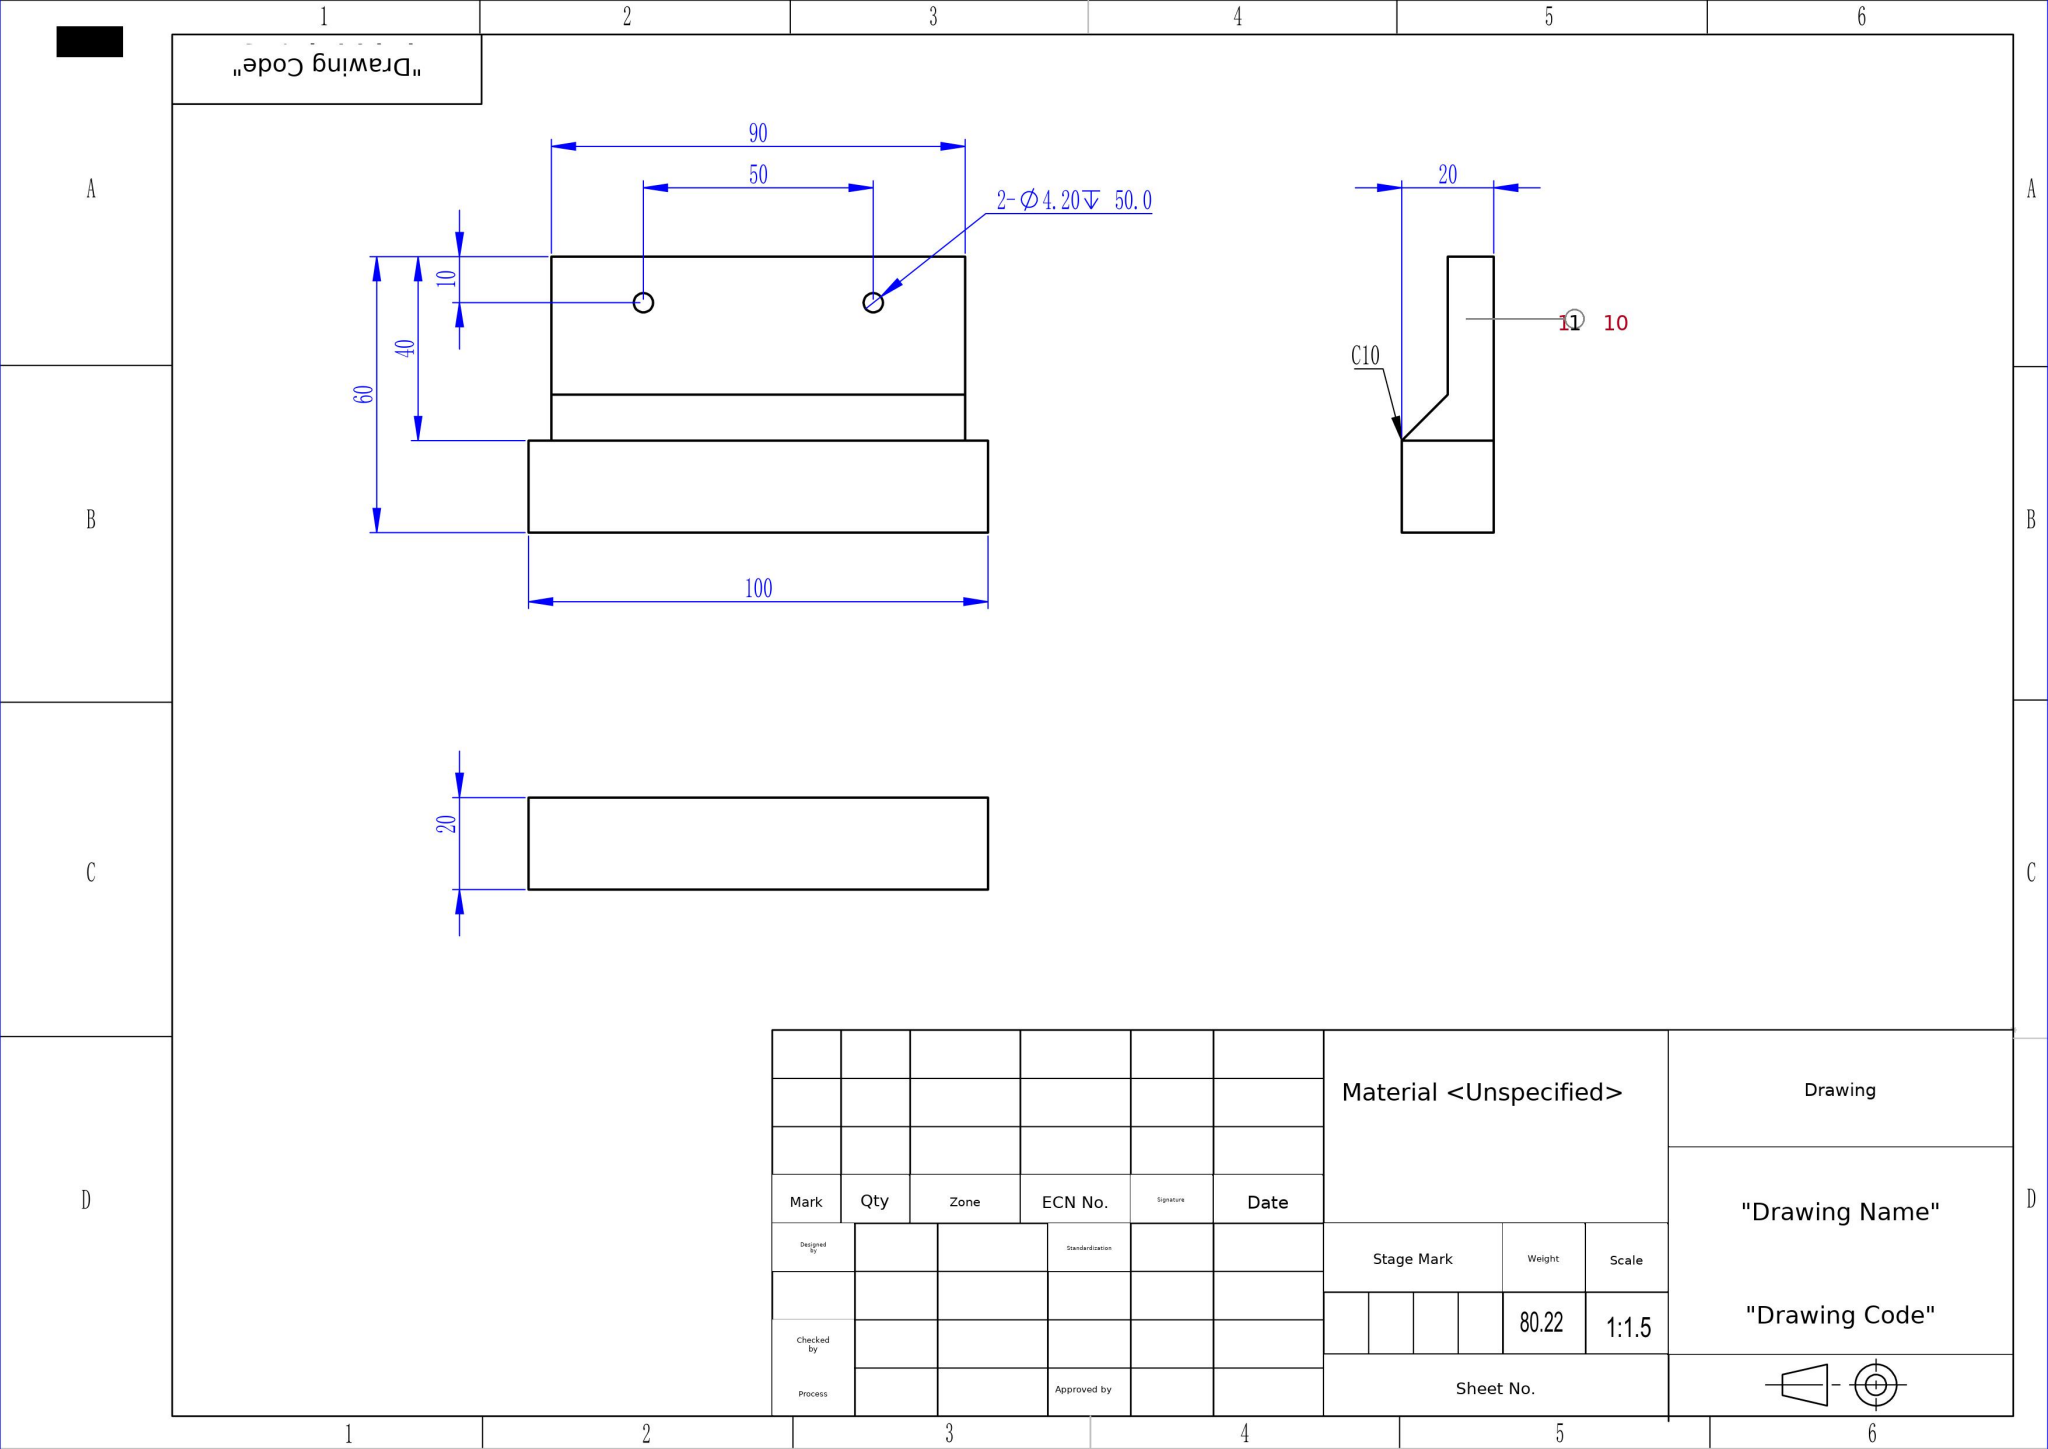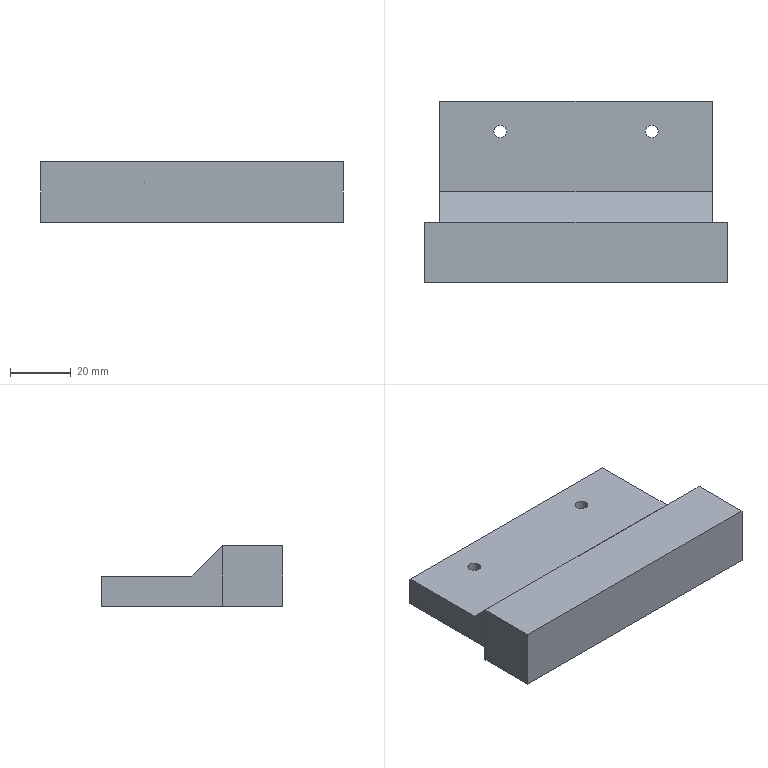Part | SolidWorks | mm | material Unspecified | 1 solid | 16 faces | box 100 x 60 x 20 mm | volume 80223 mm3 | plane 12 | cylinder 4 | commonest cylinder face diameters 4.2 x4
STEP:
#1=CARTESIAN_POINT('',(-27.1,40.,-10.));
#2=VERTEX_POINT('',#1);
#3=CARTESIAN_POINT('',(-22.9,40.,-10.));
#4=VERTEX_POINT('',#3);
#5=CARTESIAN_POINT('',(-25.,40.,-10.));
#6=DIRECTION('',(0.,0.,1.));
#7=DIRECTION('',(1.,0.,0.));
#8=AXIS2_PLACEMENT_3D('',#5,#6,#7);
#9=CIRCLE('',#8,2.1);
#10=EDGE_CURVE('',#2,#4,#9,.T.);
#11=ORIENTED_EDGE('',*,*,#10,.F.);
#12=CARTESIAN_POINT('',(-27.1,40.,0.));
#13=VERTEX_POINT('',#12);
#14=CARTESIAN_POINT('',(-27.1,40.,-50.));
#15=DIRECTION('',(0.,0.,1.));
#16=VECTOR('',#15,1000.);
#17=LINE('',#14,#16);
#18=EDGE_CURVE('',#2,#13,#17,.T.);
#19=ORIENTED_EDGE('',*,*,#18,.T.);
#20=CARTESIAN_POINT('',(-22.9,40.,0.));
#21=VERTEX_POINT('',#20);
#22=CARTESIAN_POINT('',(-25.,40.,0.));
#23=DIRECTION('',(0.,0.,1.));
#24=DIRECTION('',(1.,0.,0.));
#25=AXIS2_PLACEMENT_3D('',#22,#23,#24);
#26=CIRCLE('',#25,2.1);
#27=EDGE_CURVE('',#13,#21,#26,.T.);
#28=ORIENTED_EDGE('',*,*,#27,.T.);
#29=CARTESIAN_POINT('',(-22.9,40.,-50.));
#30=DIRECTION('',(0.,0.,1.));
#31=VECTOR('',#30,1000.);
#32=LINE('',#29,#31);
#33=EDGE_CURVE('',#4,#21,#32,.T.);
#34=ORIENTED_EDGE('',*,*,#33,.F.);
#35=EDGE_LOOP('',(#11,#19,#28,#34));
#36=FACE_OUTER_BOUND('',#35,.T.);
#37=CARTESIAN_POINT('',(-25.,40.,-50.));
#38=DIRECTION('',(0.,0.,1.));
#39=DIRECTION('',(1.,0.,0.));
#40=AXIS2_PLACEMENT_3D('',#37,#38,#39);
#41=CYLINDRICAL_SURFACE('',#40,2.1);
#42=ADVANCED_FACE('',(#36),#41,.F.);
#43=CARTESIAN_POINT('',(22.9,40.,-10.));
#44=VERTEX_POINT('',#43);
#45=CARTESIAN_POINT('',(27.1,40.,-10.));
#46=VERTEX_POINT('',#45);
#47=CARTESIAN_POINT('',(25.,40.,-10.));
#48=DIRECTION('',(0.,0.,1.));
#49=DIRECTION('',(1.,0.,0.));
#50=AXIS2_PLACEMENT_3D('',#47,#48,#49);
#51=CIRCLE('',#50,2.1);
#52=EDGE_CURVE('',#44,#46,#51,.T.);
#53=ORIENTED_EDGE('',*,*,#52,.F.);
#54=CARTESIAN_POINT('',(22.9,40.,0.));
#55=VERTEX_POINT('',#54);
#56=CARTESIAN_POINT('',(22.9,40.,-50.));
#57=DIRECTION('',(0.,0.,1.));
#58=VECTOR('',#57,1000.);
#59=LINE('',#56,#58);
#60=EDGE_CURVE('',#44,#55,#59,.T.);
#61=ORIENTED_EDGE('',*,*,#60,.T.);
#62=CARTESIAN_POINT('',(27.1,40.,0.));
#63=VERTEX_POINT('',#62);
#64=CARTESIAN_POINT('',(25.,40.,0.));
#65=DIRECTION('',(0.,0.,1.));
#66=DIRECTION('',(1.,0.,0.));
#67=AXIS2_PLACEMENT_3D('',#64,#65,#66);
#68=CIRCLE('',#67,2.1);
#69=EDGE_CURVE('',#55,#63,#68,.T.);
#70=ORIENTED_EDGE('',*,*,#69,.T.);
#71=CARTESIAN_POINT('',(27.1,40.,-50.));
#72=DIRECTION('',(0.,0.,1.));
#73=VECTOR('',#72,1000.);
#74=LINE('',#71,#73);
#75=EDGE_CURVE('',#46,#63,#74,.T.);
#76=ORIENTED_EDGE('',*,*,#75,.F.);
#77=EDGE_LOOP('',(#53,#61,#70,#76));
#78=FACE_OUTER_BOUND('',#77,.T.);
#79=CARTESIAN_POINT('',(25.,40.,-50.));
#80=DIRECTION('',(0.,0.,1.));
#81=DIRECTION('',(1.,0.,0.));
#82=AXIS2_PLACEMENT_3D('',#79,#80,#81);
#83=CYLINDRICAL_SURFACE('',#82,2.1);
#84=ADVANCED_FACE('',(#78),#83,.F.);
#85=CARTESIAN_POINT('',(45.,10.,10.));
#86=VERTEX_POINT('',#85);
#87=CARTESIAN_POINT('',(45.,10.,-10.));
#88=VERTEX_POINT('',#87);
#89=CARTESIAN_POINT('',(45.,10.,-10.));
#90=DIRECTION('',(0.,0.,-1.));
#91=VECTOR('',#90,1000.);
#92=LINE('',#89,#91);
#93=EDGE_CURVE('',#86,#88,#92,.T.);
#94=ORIENTED_EDGE('',*,*,#93,.F.);
#95=CARTESIAN_POINT('',(50.,10.,10.));
#96=VERTEX_POINT('',#95);
#97=CARTESIAN_POINT('',(-50.,10.,10.));
#98=DIRECTION('',(-1.,0.,0.));
#99=VECTOR('',#98,1000.);
#100=LINE('',#97,#99);
#101=EDGE_CURVE('',#96,#86,#100,.T.);
#102=ORIENTED_EDGE('',*,*,#101,.F.);
#103=CARTESIAN_POINT('',(50.,10.,-10.));
#104=VERTEX_POINT('',#103);
#105=CARTESIAN_POINT('',(50.,10.,-10.));
#106=DIRECTION('',(0.,0.,1.));
#107=VECTOR('',#106,1000.);
#108=LINE('',#105,#107);
#109=EDGE_CURVE('',#104,#96,#108,.T.);
#110=ORIENTED_EDGE('',*,*,#109,.F.);
#111=CARTESIAN_POINT('',(-50.,10.,-10.));
#112=DIRECTION('',(-1.,0.,0.));
#113=VECTOR('',#112,1000.);
#114=LINE('',#111,#113);
#115=EDGE_CURVE('',#104,#88,#114,.T.);
#116=ORIENTED_EDGE('',*,*,#115,.T.);
#117=EDGE_LOOP('',(#94,#102,#110,#116));
#118=FACE_OUTER_BOUND('',#117,.T.);
#119=CARTESIAN_POINT('',(-50.,10.,-10.));
#120=DIRECTION('',(0.,1.,0.));
#121=DIRECTION('',(0.,0.,1.));
#122=AXIS2_PLACEMENT_3D('',#119,#120,#121);
#123=PLANE('',#122);
#124=ADVANCED_FACE('',(#118),#123,.T.);
#125=ORIENTED_EDGE('',*,*,#109,.T.);
#126=CARTESIAN_POINT('',(50.,-10.,10.));
#127=VERTEX_POINT('',#126);
#128=CARTESIAN_POINT('',(50.,10.,10.));
#129=DIRECTION('',(0.,1.,0.));
#130=VECTOR('',#129,1000.);
#131=LINE('',#128,#130);
#132=EDGE_CURVE('',#127,#96,#131,.T.);
#133=ORIENTED_EDGE('',*,*,#132,.F.);
#134=CARTESIAN_POINT('',(50.,-10.,-10.));
#135=VERTEX_POINT('',#134);
#136=CARTESIAN_POINT('',(50.,-10.,-10.));
#137=DIRECTION('',(0.,0.,1.));
#138=VECTOR('',#137,1000.);
#139=LINE('',#136,#138);
#140=EDGE_CURVE('',#135,#127,#139,.T.);
#141=ORIENTED_EDGE('',*,*,#140,.F.);
#142=CARTESIAN_POINT('',(50.,10.,-10.));
#143=DIRECTION('',(0.,1.,0.));
#144=VECTOR('',#143,1000.);
#145=LINE('',#142,#144);
#146=EDGE_CURVE('',#135,#104,#145,.T.);
#147=ORIENTED_EDGE('',*,*,#146,.T.);
#148=EDGE_LOOP('',(#125,#133,#141,#147));
#149=FACE_OUTER_BOUND('',#148,.T.);
#150=CARTESIAN_POINT('',(50.,10.,-10.));
#151=DIRECTION('',(1.,0.,0.));
#152=DIRECTION('',(0.,0.,-1.));
#153=AXIS2_PLACEMENT_3D('',#150,#151,#152);
#154=PLANE('',#153);
#155=ADVANCED_FACE('',(#149),#154,.T.);
#156=ORIENTED_EDGE('',*,*,#140,.T.);
#157=CARTESIAN_POINT('',(-50.,-10.,10.));
#158=VERTEX_POINT('',#157);
#159=CARTESIAN_POINT('',(-50.,-10.,10.));
#160=DIRECTION('',(1.,0.,0.));
#161=VECTOR('',#160,1000.);
#162=LINE('',#159,#161);
#163=EDGE_CURVE('',#158,#127,#162,.T.);
#164=ORIENTED_EDGE('',*,*,#163,.F.);
#165=CARTESIAN_POINT('',(-50.,-10.,-10.));
#166=VERTEX_POINT('',#165);
#167=CARTESIAN_POINT('',(-50.,-10.,-10.));
#168=DIRECTION('',(0.,0.,1.));
#169=VECTOR('',#168,1000.);
#170=LINE('',#167,#169);
#171=EDGE_CURVE('',#166,#158,#170,.T.);
#172=ORIENTED_EDGE('',*,*,#171,.F.);
#173=CARTESIAN_POINT('',(-50.,-10.,-10.));
#174=DIRECTION('',(1.,0.,0.));
#175=VECTOR('',#174,1000.);
#176=LINE('',#173,#175);
#177=EDGE_CURVE('',#166,#135,#176,.T.);
#178=ORIENTED_EDGE('',*,*,#177,.T.);
#179=EDGE_LOOP('',(#156,#164,#172,#178));
#180=FACE_OUTER_BOUND('',#179,.T.);
#181=CARTESIAN_POINT('',(-50.,-10.,-10.));
#182=DIRECTION('',(0.,-1.,0.));
#183=DIRECTION('',(0.,0.,-1.));
#184=AXIS2_PLACEMENT_3D('',#181,#182,#183);
#185=PLANE('',#184);
#186=ADVANCED_FACE('',(#180),#185,.T.);
#187=ORIENTED_EDGE('',*,*,#171,.T.);
#188=CARTESIAN_POINT('',(-50.,10.,10.));
#189=VERTEX_POINT('',#188);
#190=CARTESIAN_POINT('',(-50.,10.,10.));
#191=DIRECTION('',(0.,-1.,0.));
#192=VECTOR('',#191,1000.);
#193=LINE('',#190,#192);
#194=EDGE_CURVE('',#189,#158,#193,.T.);
#195=ORIENTED_EDGE('',*,*,#194,.F.);
#196=CARTESIAN_POINT('',(-50.,10.,-10.));
#197=VERTEX_POINT('',#196);
#198=CARTESIAN_POINT('',(-50.,10.,-10.));
#199=DIRECTION('',(0.,0.,1.));
#200=VECTOR('',#199,1000.);
#201=LINE('',#198,#200);
#202=EDGE_CURVE('',#197,#189,#201,.T.);
#203=ORIENTED_EDGE('',*,*,#202,.F.);
#204=CARTESIAN_POINT('',(-50.,10.,-10.));
#205=DIRECTION('',(0.,-1.,0.));
#206=VECTOR('',#205,1000.);
#207=LINE('',#204,#206);
#208=EDGE_CURVE('',#197,#166,#207,.T.);
#209=ORIENTED_EDGE('',*,*,#208,.T.);
#210=EDGE_LOOP('',(#187,#195,#203,#209));
#211=FACE_OUTER_BOUND('',#210,.T.);
#212=CARTESIAN_POINT('',(-50.,10.,-10.));
#213=DIRECTION('',(-1.,0.,0.));
#214=DIRECTION('',(0.,0.,1.));
#215=AXIS2_PLACEMENT_3D('',#212,#213,#214);
#216=PLANE('',#215);
#217=ADVANCED_FACE('',(#211),#216,.T.);
#218=CARTESIAN_POINT('',(-45.,10.,10.));
#219=VERTEX_POINT('',#218);
#220=CARTESIAN_POINT('',(-50.,10.,10.));
#221=DIRECTION('',(-1.,0.,0.));
#222=VECTOR('',#221,1000.);
#223=LINE('',#220,#222);
#224=EDGE_CURVE('',#219,#189,#223,.T.);
#225=ORIENTED_EDGE('',*,*,#224,.F.);
#226=CARTESIAN_POINT('',(-45.,10.,-10.));
#227=VERTEX_POINT('',#226);
#228=CARTESIAN_POINT('',(-45.,10.,-10.));
#229=DIRECTION('',(0.,0.,1.));
#230=VECTOR('',#229,1000.);
#231=LINE('',#228,#230);
#232=EDGE_CURVE('',#227,#219,#231,.T.);
#233=ORIENTED_EDGE('',*,*,#232,.F.);
#234=CARTESIAN_POINT('',(-50.,10.,-10.));
#235=DIRECTION('',(-1.,0.,0.));
#236=VECTOR('',#235,1000.);
#237=LINE('',#234,#236);
#238=EDGE_CURVE('',#227,#197,#237,.T.);
#239=ORIENTED_EDGE('',*,*,#238,.T.);
#240=ORIENTED_EDGE('',*,*,#202,.T.);
#241=EDGE_LOOP('',(#225,#233,#239,#240));
#242=FACE_OUTER_BOUND('',#241,.T.);
#243=CARTESIAN_POINT('',(-50.,10.,-10.));
#244=DIRECTION('',(0.,1.,0.));
#245=DIRECTION('',(0.,0.,1.));
#246=AXIS2_PLACEMENT_3D('',#243,#244,#245);
#247=PLANE('',#246);
#248=ADVANCED_FACE('',(#242),#247,.T.);
#249=CARTESIAN_POINT('',(-25.,40.,-10.));
#250=DIRECTION('',(0.,0.,1.));
#251=DIRECTION('',(1.,0.,0.));
#252=AXIS2_PLACEMENT_3D('',#249,#250,#251);
#253=CIRCLE('',#252,2.1);
#254=EDGE_CURVE('',#4,#2,#253,.T.);
#255=ORIENTED_EDGE('',*,*,#254,.T.);
#256=ORIENTED_EDGE('',*,*,#10,.T.);
#257=EDGE_LOOP('',(#255,#256));
#258=FACE_BOUND('',#257,.T.);
#259=CARTESIAN_POINT('',(25.,40.,-10.));
#260=DIRECTION('',(0.,0.,1.));
#261=DIRECTION('',(1.,0.,0.));
#262=AXIS2_PLACEMENT_3D('',#259,#260,#261);
#263=CIRCLE('',#262,2.1);
#264=EDGE_CURVE('',#46,#44,#263,.T.);
#265=ORIENTED_EDGE('',*,*,#264,.T.);
#266=ORIENTED_EDGE('',*,*,#52,.T.);
#267=EDGE_LOOP('',(#265,#266));
#268=FACE_BOUND('',#267,.T.);
#269=CARTESIAN_POINT('',(-45.,50.,-10.));
#270=VERTEX_POINT('',#269);
#271=CARTESIAN_POINT('',(-45.,60.,-10.));
#272=DIRECTION('',(0.,-1.,0.));
#273=VECTOR('',#272,1000.);
#274=LINE('',#271,#273);
#275=EDGE_CURVE('',#270,#227,#274,.T.);
#276=ORIENTED_EDGE('',*,*,#275,.F.);
#277=CARTESIAN_POINT('',(45.,50.,-10.));
#278=VERTEX_POINT('',#277);
#279=CARTESIAN_POINT('',(0.,50.,-10.));
#280=DIRECTION('',(1.,0.,0.));
#281=VECTOR('',#280,1000.);
#282=LINE('',#279,#281);
#283=EDGE_CURVE('',#270,#278,#282,.T.);
#284=ORIENTED_EDGE('',*,*,#283,.T.);
#285=CARTESIAN_POINT('',(45.,60.,-10.));
#286=DIRECTION('',(0.,-1.,0.));
#287=VECTOR('',#286,1000.);
#288=LINE('',#285,#287);
#289=EDGE_CURVE('',#278,#88,#288,.T.);
#290=ORIENTED_EDGE('',*,*,#289,.T.);
#291=ORIENTED_EDGE('',*,*,#115,.F.);
#292=ORIENTED_EDGE('',*,*,#146,.F.);
#293=ORIENTED_EDGE('',*,*,#177,.F.);
#294=ORIENTED_EDGE('',*,*,#208,.F.);
#295=ORIENTED_EDGE('',*,*,#238,.F.);
#296=EDGE_LOOP('',(#276,#284,#290,#291,#292,#293,#294,#295));
#297=FACE_OUTER_BOUND('',#296,.T.);
#298=CARTESIAN_POINT('',(0.,0.,-10.));
#299=DIRECTION('',(0.,0.,1.));
#300=DIRECTION('',(1.,0.,0.));
#301=AXIS2_PLACEMENT_3D('',#298,#299,#300);
#302=PLANE('',#301);
#303=ADVANCED_FACE('',(#258,#268,#297),#302,.F.);
#304=ORIENTED_EDGE('',*,*,#132,.T.);
#305=ORIENTED_EDGE('',*,*,#101,.T.);
#306=CARTESIAN_POINT('',(-50.,10.,10.));
#307=DIRECTION('',(-1.,0.,0.));
#308=VECTOR('',#307,1000.);
#309=LINE('',#306,#308);
#310=EDGE_CURVE('',#86,#219,#309,.T.);
#311=ORIENTED_EDGE('',*,*,#310,.T.);
#312=ORIENTED_EDGE('',*,*,#224,.T.);
#313=ORIENTED_EDGE('',*,*,#194,.T.);
#314=ORIENTED_EDGE('',*,*,#163,.T.);
#315=EDGE_LOOP('',(#304,#305,#311,#312,#313,#314));
#316=FACE_OUTER_BOUND('',#315,.T.);
#317=CARTESIAN_POINT('',(0.,0.,10.));
#318=DIRECTION('',(0.,0.,1.));
#319=DIRECTION('',(1.,0.,0.));
#320=AXIS2_PLACEMENT_3D('',#317,#318,#319);
#321=PLANE('',#320);
#322=ADVANCED_FACE('',(#316),#321,.T.);
#323=CARTESIAN_POINT('',(-45.,50.,0.));
#324=VERTEX_POINT('',#323);
#325=CARTESIAN_POINT('',(-45.,20.,0.));
#326=VERTEX_POINT('',#325);
#327=CARTESIAN_POINT('',(-45.,60.,0.));
#328=DIRECTION('',(0.,-1.,0.));
#329=VECTOR('',#328,1000.);
#330=LINE('',#327,#329);
#331=EDGE_CURVE('',#324,#326,#330,.T.);
#332=ORIENTED_EDGE('',*,*,#331,.F.);
#333=CARTESIAN_POINT('',(-45.,50.,-50.));
#334=DIRECTION('',(0.,0.,1.));
#335=VECTOR('',#334,1000.);
#336=LINE('',#333,#335);
#337=EDGE_CURVE('',#270,#324,#336,.T.);
#338=ORIENTED_EDGE('',*,*,#337,.F.);
#339=ORIENTED_EDGE('',*,*,#275,.T.);
#340=ORIENTED_EDGE('',*,*,#232,.T.);
#341=CARTESIAN_POINT('',(-45.,45.,-25.));
#342=DIRECTION('',(0.,0.7071,-0.7071));
#343=VECTOR('',#342,1000.);
#344=LINE('',#341,#343);
#345=EDGE_CURVE('',#219,#326,#344,.T.);
#346=ORIENTED_EDGE('',*,*,#345,.T.);
#347=EDGE_LOOP('',(#332,#338,#339,#340,#346));
#348=FACE_OUTER_BOUND('',#347,.T.);
#349=CARTESIAN_POINT('',(-45.,60.,-10.));
#350=DIRECTION('',(1.,0.,0.));
#351=DIRECTION('',(0.,0.,-1.));
#352=AXIS2_PLACEMENT_3D('',#349,#350,#351);
#353=PLANE('',#352);
#354=ADVANCED_FACE('',(#348),#353,.F.);
#355=CARTESIAN_POINT('',(-25.,40.,0.));
#356=DIRECTION('',(0.,0.,1.));
#357=DIRECTION('',(1.,0.,0.));
#358=AXIS2_PLACEMENT_3D('',#355,#356,#357);
#359=CIRCLE('',#358,2.1);
#360=EDGE_CURVE('',#21,#13,#359,.T.);
#361=ORIENTED_EDGE('',*,*,#360,.F.);
#362=ORIENTED_EDGE('',*,*,#27,.F.);
#363=EDGE_LOOP('',(#361,#362));
#364=FACE_BOUND('',#363,.T.);
#365=CARTESIAN_POINT('',(25.,40.,0.));
#366=DIRECTION('',(0.,0.,1.));
#367=DIRECTION('',(1.,0.,0.));
#368=AXIS2_PLACEMENT_3D('',#365,#366,#367);
#369=CIRCLE('',#368,2.1);
#370=EDGE_CURVE('',#63,#55,#369,.T.);
#371=ORIENTED_EDGE('',*,*,#370,.F.);
#372=ORIENTED_EDGE('',*,*,#69,.F.);
#373=EDGE_LOOP('',(#371,#372));
#374=FACE_BOUND('',#373,.T.);
#375=CARTESIAN_POINT('',(45.,50.,0.));
#376=VERTEX_POINT('',#375);
#377=CARTESIAN_POINT('',(45.,20.,0.));
#378=VERTEX_POINT('',#377);
#379=CARTESIAN_POINT('',(45.,60.,0.));
#380=DIRECTION('',(0.,-1.,0.));
#381=VECTOR('',#380,1000.);
#382=LINE('',#379,#381);
#383=EDGE_CURVE('',#376,#378,#382,.T.);
#384=ORIENTED_EDGE('',*,*,#383,.F.);
#385=CARTESIAN_POINT('',(-45.,50.,0.));
#386=DIRECTION('',(1.,0.,0.));
#387=VECTOR('',#386,1000.);
#388=LINE('',#385,#387);
#389=EDGE_CURVE('',#324,#376,#388,.T.);
#390=ORIENTED_EDGE('',*,*,#389,.F.);
#391=ORIENTED_EDGE('',*,*,#331,.T.);
#392=CARTESIAN_POINT('',(-45.,20.,0.));
#393=DIRECTION('',(1.,0.,0.));
#394=VECTOR('',#393,1000.);
#395=LINE('',#392,#394);
#396=EDGE_CURVE('',#326,#378,#395,.T.);
#397=ORIENTED_EDGE('',*,*,#396,.T.);
#398=EDGE_LOOP('',(#384,#390,#391,#397));
#399=FACE_OUTER_BOUND('',#398,.T.);
#400=CARTESIAN_POINT('',(-45.,60.,0.));
#401=DIRECTION('',(0.,0.,-1.));
#402=DIRECTION('',(-1.,0.,0.));
#403=AXIS2_PLACEMENT_3D('',#400,#401,#402);
#404=PLANE('',#403);
#405=ADVANCED_FACE('',(#364,#374,#399),#404,.F.);
#406=ORIENTED_EDGE('',*,*,#289,.F.);
#407=CARTESIAN_POINT('',(45.,50.,-50.));
#408=DIRECTION('',(0.,0.,1.));
#409=VECTOR('',#408,1000.);
#410=LINE('',#407,#409);
#411=EDGE_CURVE('',#278,#376,#410,.T.);
#412=ORIENTED_EDGE('',*,*,#411,.T.);
#413=ORIENTED_EDGE('',*,*,#383,.T.);
#414=CARTESIAN_POINT('',(45.,45.,-25.));
#415=DIRECTION('',(-0.,-0.7071,0.7071));
#416=VECTOR('',#415,1000.);
#417=LINE('',#414,#416);
#418=EDGE_CURVE('',#378,#86,#417,.T.);
#419=ORIENTED_EDGE('',*,*,#418,.T.);
#420=ORIENTED_EDGE('',*,*,#93,.T.);
#421=EDGE_LOOP('',(#406,#412,#413,#419,#420));
#422=FACE_OUTER_BOUND('',#421,.T.);
#423=CARTESIAN_POINT('',(45.,60.,-10.));
#424=DIRECTION('',(-1.,0.,-0.));
#425=DIRECTION('',(-0.,0.,1.));
#426=AXIS2_PLACEMENT_3D('',#423,#424,#425);
#427=PLANE('',#426);
#428=ADVANCED_FACE('',(#422),#427,.F.);
#429=ORIENTED_EDGE('',*,*,#345,.F.);
#430=ORIENTED_EDGE('',*,*,#310,.F.);
#431=ORIENTED_EDGE('',*,*,#418,.F.);
#432=ORIENTED_EDGE('',*,*,#396,.F.);
#433=EDGE_LOOP('',(#429,#430,#431,#432));
#434=FACE_OUTER_BOUND('',#433,.T.);
#435=CARTESIAN_POINT('',(-45.,20.,0.));
#436=DIRECTION('',(0.,-0.7071,-0.7071));
#437=DIRECTION('',(1.,0.,0.));
#438=AXIS2_PLACEMENT_3D('',#435,#436,#437);
#439=PLANE('',#438);
#440=ADVANCED_FACE('',(#434),#439,.F.);
#441=ORIENTED_EDGE('',*,*,#337,.T.);
#442=ORIENTED_EDGE('',*,*,#389,.T.);
#443=ORIENTED_EDGE('',*,*,#411,.F.);
#444=ORIENTED_EDGE('',*,*,#283,.F.);
#445=EDGE_LOOP('',(#441,#442,#443,#444));
#446=FACE_OUTER_BOUND('',#445,.T.);
#447=CARTESIAN_POINT('',(-45.,50.,-50.));
#448=DIRECTION('',(0.,-1.,0.));
#449=DIRECTION('',(0.,0.,-1.));
#450=AXIS2_PLACEMENT_3D('',#447,#448,#449);
#451=PLANE('',#450);
#452=ADVANCED_FACE('',(#446),#451,.F.);
#453=ORIENTED_EDGE('',*,*,#60,.F.);
#454=ORIENTED_EDGE('',*,*,#264,.F.);
#455=ORIENTED_EDGE('',*,*,#75,.T.);
#456=ORIENTED_EDGE('',*,*,#370,.T.);
#457=EDGE_LOOP('',(#453,#454,#455,#456));
#458=FACE_OUTER_BOUND('',#457,.T.);
#459=CARTESIAN_POINT('',(25.,40.,-50.));
#460=DIRECTION('',(0.,0.,1.));
#461=DIRECTION('',(1.,0.,0.));
#462=AXIS2_PLACEMENT_3D('',#459,#460,#461);
#463=CYLINDRICAL_SURFACE('',#462,2.1);
#464=ADVANCED_FACE('',(#458),#463,.F.);
#465=ORIENTED_EDGE('',*,*,#18,.F.);
#466=ORIENTED_EDGE('',*,*,#254,.F.);
#467=ORIENTED_EDGE('',*,*,#33,.T.);
#468=ORIENTED_EDGE('',*,*,#360,.T.);
#469=EDGE_LOOP('',(#465,#466,#467,#468));
#470=FACE_OUTER_BOUND('',#469,.T.);
#471=CARTESIAN_POINT('',(-25.,40.,-50.));
#472=DIRECTION('',(0.,0.,1.));
#473=DIRECTION('',(1.,0.,0.));
#474=AXIS2_PLACEMENT_3D('',#471,#472,#473);
#475=CYLINDRICAL_SURFACE('',#474,2.1);
#476=ADVANCED_FACE('',(#470),#475,.F.);
#477=CLOSED_SHELL('',(#42,#84,#124,#155,#186,#217,#248,#303,#322,#354,#405,#428,#440,#452,#464,#476));
#478=MANIFOLD_SOLID_BREP('',#477);
#479=CARTESIAN_POINT('',(0.,0.,0.));
#480=DIRECTION('',(0.,0.,1.));
#481=DIRECTION('',(1.,0.,0.));
#482=AXIS2_PLACEMENT_3D('',#479,#480,#481);
#483=(LENGTH_UNIT()NAMED_UNIT(*)SI_UNIT(.MILLI.,.METRE.));
#484=UNCERTAINTY_MEASURE_WITH_UNIT(LENGTH_MEASURE(0.00001),#483,'','');
#485=(NAMED_UNIT(*)PLANE_ANGLE_UNIT()SI_UNIT($,.RADIAN.));
#486=(NAMED_UNIT(*)SI_UNIT($,.STERADIAN.)SOLID_ANGLE_UNIT());
#487=(GEOMETRIC_REPRESENTATION_CONTEXT(3)GLOBAL_UNCERTAINTY_ASSIGNED_CONTEXT((#484))GLOBAL_UNIT_ASSIGNED_CONTEXT((#483,#485,#486))REPRESENTATION_CONTEXT('',''));
#488=ADVANCED_BREP_SHAPE_REPRESENTATION('',(#478,#482),#487);